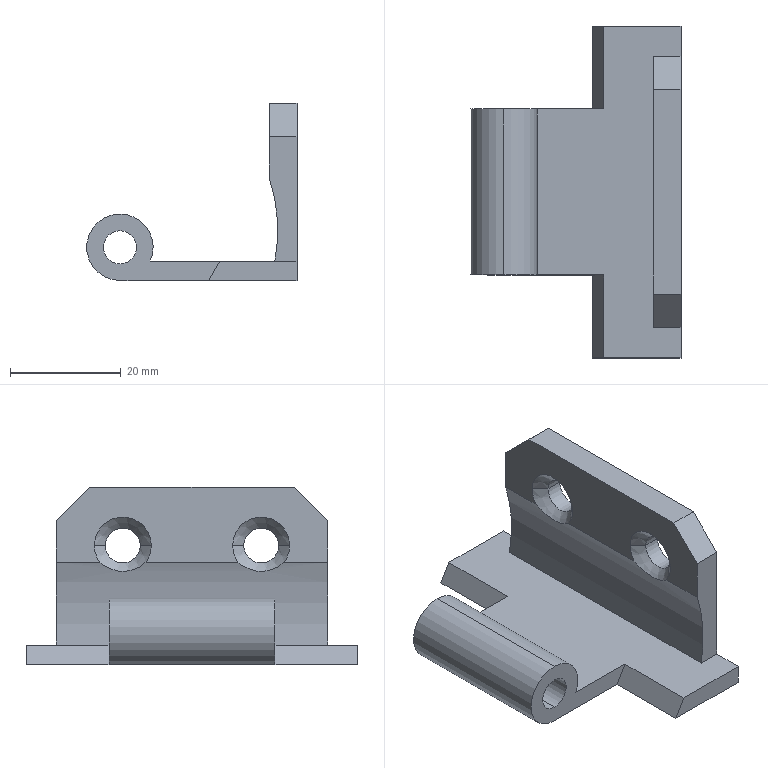Component | SolidWorks | SidePanelAssembly-1_GL213-1Hinge2-4 | 1 solid | 28 faces | box 38 x 60 x 32 mm | volume 12628 mm3 | plane 15 | cylinder 9 | cone 4 | commonest cylinder face diameters 6.3 x4 6 x2 12 x2 60 x1
build123d program:
from build123d import *

# Parameters (mm, degrees)
BOSS_EXTRUDE1_DEPTH = 60
SKETCH2_W           = 49
SKETCH2_H           = 5
BOSS_EXTRUDE2_DEPTH = 28.5
SKETCH3_W           = 3.5
SKETCH3_H           = 30
BOSS_EXTRUDE3_DEPTH = 27
SKETCH4_R           = 6
BOSS_EXTRUDE4_DEPTH = 30
SKETCH5_R           = 3
CUT_EXTRUDE1_DEPTH  = 30
SKETCH6_R           = 3.15
CUT_EXTRUDE2_DEPTH  = 30
CHAMFER1_SIZE       = 2
CHAMFER2_SIZE       = 6
CUT_EXTRUDE3_DEPTH  = 74.744


with BuildPart() as part:
    # Sketch1 → Boss-Extrude1 (new body)
    with BuildSketch(Plane.XY):
        Polygon((0, 0), (3.5, 0), (3.5, 13.979), (0, 16), align=None)
    extrude(amount=BOSS_EXTRUDE1_DEPTH)

    # Sketch2 → Boss-Extrude2 (add)
    with BuildSketch(Plane(origin=(3.5, 0, 0), x_dir=(0, 0, -1), z_dir=(1, 0, 0))):
        with Locations((-30, 2.5)):
            Rectangle(SKETCH2_W, SKETCH2_H)
    extrude(amount=BOSS_EXTRUDE2_DEPTH)

    # Sketch3 → Boss-Extrude3 (add)
    with BuildSketch(Plane(origin=(0, 5, 0), x_dir=(1, 0, 0), z_dir=(0, 1, 0))):
        with Locations((1.75, -30)):
            Rectangle(SKETCH3_W, SKETCH3_H)
    extrude(amount=BOSS_EXTRUDE3_DEPTH)

    # Sketch4 → Boss-Extrude4 (add)
    with BuildSketch(Plane.XY.offset(45)):
        with Locations((6, 32)):
            Circle(SKETCH4_R)
    extrude(amount=-BOSS_EXTRUDE4_DEPTH)

    # Sketch5 → Cut-Extrude1 (cut)
    with BuildSketch(Plane.XY.offset(45)):
        with Locations((6, 32)):
            Circle(SKETCH5_R)
    extrude(amount=-CUT_EXTRUDE1_DEPTH, mode=Mode.SUBTRACT)

    # Sketch6 → Cut-Extrude2 (cut)
    with BuildSketch(Plane(origin=(0, 5, 0), x_dir=(1, 0, 0), z_dir=(0, 1, 0))):
        with Locations(Location((21.5, -42.5, 0), (0, 0, 270))):
            Circle(SKETCH6_R)
        with Locations(Location((21.5, -17.5, 0), (0, 0, 270))):
            Circle(SKETCH6_R)
    extrude(amount=-CUT_EXTRUDE2_DEPTH, mode=Mode.SUBTRACT)

    # Chamfer1
    chamfer1_edges = [part.edges().sort_by_distance(p)[0] for p in [
        (21.5, 5, 39.35),
        (21.5, 5, 14.35),
    ]]
    chamfer(chamfer1_edges, length=CHAMFER1_SIZE)

    # Chamfer2
    chamfer2_edges = [part.edges().sort_by_distance(p)[0] for p in [
        (32, 2.5, 54.5),
        (32, 2.5, 5.5),
    ]]
    chamfer(chamfer2_edges, length=CHAMFER2_SIZE)

    # Sketch7 → Cut-Extrude3 (cut, through all)
    with BuildSketch(Plane.XY.offset(54.5)):
        with BuildLine():
            Line((3.5, 4), (3.5, 5))
            Line((3.5, 5), (18.5, 5))
            ThreePointArc((18.5, 5), (11.064, 3.545), (3.5, 4))
        make_face()
    extrude(amount=-CUT_EXTRUDE3_DEPTH, mode=Mode.SUBTRACT)


solid = part.part

# Placed as in the assembly
solid = solid.moved(Location((-417.218, 212.1, -600), (90, 0, 90)))
STEP:
#1=CARTESIAN_POINT('',(-16.544,7.785,-22.776));
#2=VERTEX_POINT('',#1);
#3=CARTESIAN_POINT('',(-16.544,7.537,-22.776));
#4=VERTEX_POINT('',#3);
#5=CARTESIAN_POINT('',(-16.544,7.661,-22.776));
#6=DIRECTION('',(-1.,-0.,-0.));
#7=DIRECTION('',(0.,1.,0.));
#8=AXIS2_PLACEMENT_3D('',#5,#6,#7);
#9=CIRCLE('',#8,0.124);
#10=EDGE_CURVE('',#2,#4,#9,.T.);
#11=ORIENTED_EDGE('',*,*,#10,.F.);
#12=CARTESIAN_POINT('',(-16.623,7.864,-22.776));
#13=VERTEX_POINT('',#12);
#14=CARTESIAN_POINT('',(-16.544,7.785,-22.776));
#15=DIRECTION('',(-0.7071,0.7071,-0.));
#16=VECTOR('',#15,39.37);
#17=LINE('',#14,#16);
#18=EDGE_CURVE('',#2,#13,#17,.T.);
#19=ORIENTED_EDGE('',*,*,#18,.T.);
#20=CARTESIAN_POINT('',(-16.623,7.826,-22.894));
#21=VERTEX_POINT('',#20);
#22=CARTESIAN_POINT('',(-16.623,7.661,-22.776));
#23=DIRECTION('',(1.,0.,0.));
#24=DIRECTION('',(0.,1.,0.));
#25=AXIS2_PLACEMENT_3D('',#22,#23,#24);
#26=CIRCLE('',#25,0.2028);
#27=EDGE_CURVE('',#21,#13,#26,.T.);
#28=ORIENTED_EDGE('',*,*,#27,.F.);
#29=CARTESIAN_POINT('',(-16.623,7.497,-22.894));
#30=VERTEX_POINT('',#29);
#31=CARTESIAN_POINT('',(-16.623,7.497,-22.894));
#32=CARTESIAN_POINT('',(-16.619,7.508,-22.904));
#33=CARTESIAN_POINT('',(-16.617,7.52,-22.913));
#34=CARTESIAN_POINT('',(-16.613,7.538,-22.925));
#35=CARTESIAN_POINT('',(-16.612,7.545,-22.928));
#36=CARTESIAN_POINT('',(-16.61,7.558,-22.935));
#37=CARTESIAN_POINT('',(-16.609,7.565,-22.938));
#38=CARTESIAN_POINT('',(-16.606,7.586,-22.947));
#39=CARTESIAN_POINT('',(-16.605,7.601,-22.951));
#40=CARTESIAN_POINT('',(-16.604,7.623,-22.956));
#41=CARTESIAN_POINT('',(-16.604,7.631,-22.957));
#42=CARTESIAN_POINT('',(-16.603,7.646,-22.958));
#43=CARTESIAN_POINT('',(-16.603,7.653,-22.959));
#44=CARTESIAN_POINT('',(-16.603,7.676,-22.959));
#45=CARTESIAN_POINT('',(-16.604,7.691,-22.957));
#46=CARTESIAN_POINT('',(-16.605,7.721,-22.952));
#47=CARTESIAN_POINT('',(-16.606,7.736,-22.947));
#48=CARTESIAN_POINT('',(-16.61,7.764,-22.936));
#49=CARTESIAN_POINT('',(-16.612,7.777,-22.929));
#50=CARTESIAN_POINT('',(-16.617,7.803,-22.913));
#51=CARTESIAN_POINT('',(-16.619,7.815,-22.904));
#52=CARTESIAN_POINT('',(-16.623,7.826,-22.894));
#53=B_SPLINE_CURVE_WITH_KNOTS('',3,(#31,#32,#33,#34,#35,#36,#37,#38,#39,#40,#41,#42,#43,#44,#45,#46,#47,#48,#49,#50,#51,#52),.UNSPECIFIED.,.F.,.F.,(4,2,2,2,2,2,2,2,2,2,4),(0.0003209,0.001473,0.002049,0.002625,0.003777,0.004353,0.00493,0.006082,0.007234,0.008386,0.009538),.UNSPECIFIED.);
#54=EDGE_CURVE('',#30,#21,#53,.T.);
#55=ORIENTED_EDGE('',*,*,#54,.F.);
#56=CARTESIAN_POINT('',(-16.623,7.459,-22.776));
#57=VERTEX_POINT('',#56);
#58=CARTESIAN_POINT('',(-16.623,7.661,-22.776));
#59=DIRECTION('',(1.,0.,0.));
#60=DIRECTION('',(0.,1.,0.));
#61=AXIS2_PLACEMENT_3D('',#58,#59,#60);
#62=CIRCLE('',#61,0.2028);
#63=EDGE_CURVE('',#57,#30,#62,.T.);
#64=ORIENTED_EDGE('',*,*,#63,.F.);
#65=CARTESIAN_POINT('',(-16.544,7.537,-22.776));
#66=DIRECTION('',(-0.7071,-0.7071,-0.));
#67=VECTOR('',#66,39.37);
#68=LINE('',#65,#67);
#69=EDGE_CURVE('',#4,#57,#68,.T.);
#70=ORIENTED_EDGE('',*,*,#69,.F.);
#71=EDGE_LOOP('',(#11,#19,#28,#55,#64,#70));
#72=FACE_OUTER_BOUND('',#71,.T.);
#73=CARTESIAN_POINT('',(-16.544,7.661,-22.776));
#74=DIRECTION('',(-1.,-0.,-0.));
#75=DIRECTION('',(0.,-1.,0.));
#76=AXIS2_PLACEMENT_3D('',#73,#74,#75);
#77=CONICAL_SURFACE('',#76,0.124,0.7854);
#78=ADVANCED_FACE('',(#72),#77,.F.);
#79=CARTESIAN_POINT('',(-16.544,6.801,-22.776));
#80=VERTEX_POINT('',#79);
#81=CARTESIAN_POINT('',(-16.544,6.553,-22.776));
#82=VERTEX_POINT('',#81);
#83=CARTESIAN_POINT('',(-16.544,6.677,-22.776));
#84=DIRECTION('',(-1.,-0.,-0.));
#85=DIRECTION('',(0.,1.,0.));
#86=AXIS2_PLACEMENT_3D('',#83,#84,#85);
#87=CIRCLE('',#86,0.124);
#88=EDGE_CURVE('',#80,#82,#87,.T.);
#89=ORIENTED_EDGE('',*,*,#88,.F.);
#90=CARTESIAN_POINT('',(-16.623,6.88,-22.776));
#91=VERTEX_POINT('',#90);
#92=CARTESIAN_POINT('',(-16.544,6.801,-22.776));
#93=DIRECTION('',(-0.7071,0.7071,-0.));
#94=VECTOR('',#93,39.37);
#95=LINE('',#92,#94);
#96=EDGE_CURVE('',#80,#91,#95,.T.);
#97=ORIENTED_EDGE('',*,*,#96,.T.);
#98=CARTESIAN_POINT('',(-16.623,6.842,-22.894));
#99=VERTEX_POINT('',#98);
#100=CARTESIAN_POINT('',(-16.623,6.677,-22.776));
#101=DIRECTION('',(1.,0.,0.));
#102=DIRECTION('',(0.,1.,0.));
#103=AXIS2_PLACEMENT_3D('',#100,#101,#102);
#104=CIRCLE('',#103,0.2028);
#105=EDGE_CURVE('',#99,#91,#104,.T.);
#106=ORIENTED_EDGE('',*,*,#105,.F.);
#107=CARTESIAN_POINT('',(-16.623,6.512,-22.894));
#108=VERTEX_POINT('',#107);
#109=CARTESIAN_POINT('',(-16.623,6.512,-22.894));
#110=CARTESIAN_POINT('',(-16.619,6.523,-22.904));
#111=CARTESIAN_POINT('',(-16.617,6.535,-22.913));
#112=CARTESIAN_POINT('',(-16.613,6.554,-22.925));
#113=CARTESIAN_POINT('',(-16.612,6.561,-22.928));
#114=CARTESIAN_POINT('',(-16.61,6.574,-22.935));
#115=CARTESIAN_POINT('',(-16.609,6.581,-22.938));
#116=CARTESIAN_POINT('',(-16.606,6.602,-22.947));
#117=CARTESIAN_POINT('',(-16.605,6.617,-22.951));
#118=CARTESIAN_POINT('',(-16.604,6.639,-22.956));
#119=CARTESIAN_POINT('',(-16.604,6.646,-22.957));
#120=CARTESIAN_POINT('',(-16.603,6.661,-22.958));
#121=CARTESIAN_POINT('',(-16.603,6.669,-22.959));
#122=CARTESIAN_POINT('',(-16.603,6.692,-22.959));
#123=CARTESIAN_POINT('',(-16.604,6.707,-22.957));
#124=CARTESIAN_POINT('',(-16.605,6.737,-22.952));
#125=CARTESIAN_POINT('',(-16.606,6.752,-22.947));
#126=CARTESIAN_POINT('',(-16.61,6.78,-22.936));
#127=CARTESIAN_POINT('',(-16.612,6.793,-22.929));
#128=CARTESIAN_POINT('',(-16.617,6.819,-22.913));
#129=CARTESIAN_POINT('',(-16.619,6.831,-22.904));
#130=CARTESIAN_POINT('',(-16.623,6.842,-22.894));
#131=B_SPLINE_CURVE_WITH_KNOTS('',3,(#109,#110,#111,#112,#113,#114,#115,#116,#117,#118,#119,#120,#121,#122,#123,#124,#125,#126,#127,#128,#129,#130),.UNSPECIFIED.,.F.,.F.,(4,2,2,2,2,2,2,2,2,2,4),(0.0003209,0.001473,0.002049,0.002625,0.003777,0.004353,0.00493,0.006082,0.007234,0.008386,0.009538),.UNSPECIFIED.);
#132=EDGE_CURVE('',#108,#99,#131,.T.);
#133=ORIENTED_EDGE('',*,*,#132,.F.);
#134=CARTESIAN_POINT('',(-16.623,6.474,-22.776));
#135=VERTEX_POINT('',#134);
#136=CARTESIAN_POINT('',(-16.623,6.677,-22.776));
#137=DIRECTION('',(1.,0.,0.));
#138=DIRECTION('',(0.,1.,0.));
#139=AXIS2_PLACEMENT_3D('',#136,#137,#138);
#140=CIRCLE('',#139,0.2028);
#141=EDGE_CURVE('',#135,#108,#140,.T.);
#142=ORIENTED_EDGE('',*,*,#141,.F.);
#143=CARTESIAN_POINT('',(-16.544,6.553,-22.776));
#144=DIRECTION('',(-0.7071,-0.7071,-0.));
#145=VECTOR('',#144,39.37);
#146=LINE('',#143,#145);
#147=EDGE_CURVE('',#82,#135,#146,.T.);
#148=ORIENTED_EDGE('',*,*,#147,.F.);
#149=EDGE_LOOP('',(#89,#97,#106,#133,#142,#148));
#150=FACE_OUTER_BOUND('',#149,.T.);
#151=CARTESIAN_POINT('',(-16.544,6.677,-22.776));
#152=DIRECTION('',(-1.,-0.,-0.));
#153=DIRECTION('',(0.,-1.,0.));
#154=AXIS2_PLACEMENT_3D('',#151,#152,#153);
#155=CONICAL_SURFACE('',#154,0.124,0.7854);
#156=ADVANCED_FACE('',(#150),#155,.F.);
#157=CARTESIAN_POINT('',(-16.426,7.785,-22.776));
#158=VERTEX_POINT('',#157);
#159=CARTESIAN_POINT('',(-16.426,7.537,-22.776));
#160=VERTEX_POINT('',#159);
#161=CARTESIAN_POINT('',(-16.426,7.661,-22.776));
#162=DIRECTION('',(-1.,-0.,-0.));
#163=DIRECTION('',(0.,-1.,0.));
#164=AXIS2_PLACEMENT_3D('',#161,#162,#163);
#165=CIRCLE('',#164,0.124);
#166=EDGE_CURVE('',#158,#160,#165,.T.);
#167=ORIENTED_EDGE('',*,*,#166,.F.);
#168=CARTESIAN_POINT('',(-15.442,7.785,-22.776));
#169=DIRECTION('',(-1.,-0.,-0.));
#170=VECTOR('',#169,39.37);
#171=LINE('',#168,#170);
#172=EDGE_CURVE('',#158,#2,#171,.T.);
#173=ORIENTED_EDGE('',*,*,#172,.T.);
#174=ORIENTED_EDGE('',*,*,#10,.T.);
#175=CARTESIAN_POINT('',(-15.442,7.537,-22.776));
#176=DIRECTION('',(-1.,-0.,-0.));
#177=VECTOR('',#176,39.37);
#178=LINE('',#175,#177);
#179=EDGE_CURVE('',#160,#4,#178,.T.);
#180=ORIENTED_EDGE('',*,*,#179,.F.);
#181=EDGE_LOOP('',(#167,#173,#174,#180));
#182=FACE_OUTER_BOUND('',#181,.T.);
#183=CARTESIAN_POINT('',(-15.442,7.661,-22.776));
#184=DIRECTION('',(-1.,-0.,-0.));
#185=DIRECTION('',(0.,-1.,0.));
#186=AXIS2_PLACEMENT_3D('',#183,#184,#185);
#187=CYLINDRICAL_SURFACE('',#186,0.124);
#188=ADVANCED_FACE('',(#182),#187,.F.);
#189=CARTESIAN_POINT('',(-16.426,6.801,-22.776));
#190=VERTEX_POINT('',#189);
#191=CARTESIAN_POINT('',(-16.426,6.553,-22.776));
#192=VERTEX_POINT('',#191);
#193=CARTESIAN_POINT('',(-16.426,6.677,-22.776));
#194=DIRECTION('',(-1.,-0.,-0.));
#195=DIRECTION('',(0.,-1.,0.));
#196=AXIS2_PLACEMENT_3D('',#193,#194,#195);
#197=CIRCLE('',#196,0.124);
#198=EDGE_CURVE('',#190,#192,#197,.T.);
#199=ORIENTED_EDGE('',*,*,#198,.F.);
#200=CARTESIAN_POINT('',(-15.442,6.801,-22.776));
#201=DIRECTION('',(-1.,-0.,-0.));
#202=VECTOR('',#201,39.37);
#203=LINE('',#200,#202);
#204=EDGE_CURVE('',#190,#80,#203,.T.);
#205=ORIENTED_EDGE('',*,*,#204,.T.);
#206=ORIENTED_EDGE('',*,*,#88,.T.);
#207=CARTESIAN_POINT('',(-15.442,6.553,-22.776));
#208=DIRECTION('',(-1.,-0.,-0.));
#209=VECTOR('',#208,39.37);
#210=LINE('',#207,#209);
#211=EDGE_CURVE('',#192,#82,#210,.T.);
#212=ORIENTED_EDGE('',*,*,#211,.F.);
#213=EDGE_LOOP('',(#199,#205,#206,#212));
#214=FACE_OUTER_BOUND('',#213,.T.);
#215=CARTESIAN_POINT('',(-15.442,6.677,-22.776));
#216=DIRECTION('',(-1.,-0.,-0.));
#217=DIRECTION('',(0.,-1.,0.));
#218=AXIS2_PLACEMENT_3D('',#215,#216,#217);
#219=CYLINDRICAL_SURFACE('',#218,0.124);
#220=ADVANCED_FACE('',(#214),#219,.F.);
#221=CARTESIAN_POINT('',(-17.686,7.76,-23.504));
#222=VERTEX_POINT('',#221);
#223=CARTESIAN_POINT('',(-17.686,7.76,-23.268));
#224=VERTEX_POINT('',#223);
#225=CARTESIAN_POINT('',(-17.686,7.76,-23.386));
#226=DIRECTION('',(0.,-1.,-0.));
#227=DIRECTION('',(0.,0.,1.));
#228=AXIS2_PLACEMENT_3D('',#225,#226,#227);
#229=CIRCLE('',#228,0.1181);
#230=EDGE_CURVE('',#222,#224,#229,.T.);
#231=ORIENTED_EDGE('',*,*,#230,.F.);
#232=CARTESIAN_POINT('',(-17.686,6.579,-23.504));
#233=VERTEX_POINT('',#232);
#234=CARTESIAN_POINT('',(-17.686,7.76,-23.504));
#235=DIRECTION('',(0.,-1.,-0.));
#236=VECTOR('',#235,39.37);
#237=LINE('',#234,#236);
#238=EDGE_CURVE('',#222,#233,#237,.T.);
#239=ORIENTED_EDGE('',*,*,#238,.T.);
#240=CARTESIAN_POINT('',(-17.686,6.579,-23.268));
#241=VERTEX_POINT('',#240);
#242=CARTESIAN_POINT('',(-17.686,6.579,-23.386));
#243=DIRECTION('',(0.,-1.,-0.));
#244=DIRECTION('',(0.,0.,1.));
#245=AXIS2_PLACEMENT_3D('',#242,#243,#244);
#246=CIRCLE('',#245,0.1181);
#247=EDGE_CURVE('',#233,#241,#246,.T.);
#248=ORIENTED_EDGE('',*,*,#247,.T.);
#249=CARTESIAN_POINT('',(-17.686,7.76,-23.268));
#250=DIRECTION('',(0.,-1.,-0.));
#251=VECTOR('',#250,39.37);
#252=LINE('',#249,#251);
#253=EDGE_CURVE('',#224,#241,#252,.T.);
#254=ORIENTED_EDGE('',*,*,#253,.F.);
#255=EDGE_LOOP('',(#231,#239,#248,#254));
#256=FACE_OUTER_BOUND('',#255,.T.);
#257=CARTESIAN_POINT('',(-17.686,7.76,-23.386));
#258=DIRECTION('',(0.,-1.,-0.));
#259=DIRECTION('',(0.,0.,1.));
#260=AXIS2_PLACEMENT_3D('',#257,#258,#259);
#261=CYLINDRICAL_SURFACE('',#260,0.1181);
#262=ADVANCED_FACE('',(#256),#261,.F.);
#263=CARTESIAN_POINT('',(-17.471,7.76,-23.484));
#264=VERTEX_POINT('',#263);
#265=CARTESIAN_POINT('',(-17.686,7.76,-23.15));
#266=VERTEX_POINT('',#265);
#267=CARTESIAN_POINT('',(-17.686,7.76,-23.386));
#268=DIRECTION('',(0.,-1.,-0.));
#269=DIRECTION('',(0.,0.,1.));
#270=AXIS2_PLACEMENT_3D('',#267,#268,#269);
#271=CIRCLE('',#270,0.2362);
#272=EDGE_CURVE('',#264,#266,#271,.T.);
#273=ORIENTED_EDGE('',*,*,#272,.T.);
#274=CARTESIAN_POINT('',(-17.686,6.579,-23.15));
#275=VERTEX_POINT('',#274);
#276=CARTESIAN_POINT('',(-17.686,7.76,-23.15));
#277=DIRECTION('',(0.,-1.,-0.));
#278=VECTOR('',#277,39.37);
#279=LINE('',#276,#278);
#280=EDGE_CURVE('',#266,#275,#279,.T.);
#281=ORIENTED_EDGE('',*,*,#280,.T.);
#282=CARTESIAN_POINT('',(-17.471,6.579,-23.484));
#283=VERTEX_POINT('',#282);
#284=CARTESIAN_POINT('',(-17.686,6.579,-23.386));
#285=DIRECTION('',(0.,-1.,-0.));
#286=DIRECTION('',(0.,0.,1.));
#287=AXIS2_PLACEMENT_3D('',#284,#285,#286);
#288=CIRCLE('',#287,0.2362);
#289=EDGE_CURVE('',#283,#275,#288,.T.);
#290=ORIENTED_EDGE('',*,*,#289,.F.);
#291=CARTESIAN_POINT('',(-17.471,7.76,-23.484));
#292=DIRECTION('',(0.,-1.,-0.));
#293=VECTOR('',#292,39.37);
#294=LINE('',#291,#293);
#295=EDGE_CURVE('',#264,#283,#294,.T.);
#296=ORIENTED_EDGE('',*,*,#295,.F.);
#297=EDGE_LOOP('',(#273,#281,#290,#296));
#298=FACE_OUTER_BOUND('',#297,.T.);
#299=CARTESIAN_POINT('',(-17.686,7.76,-23.386));
#300=DIRECTION('',(0.,-1.,-0.));
#301=DIRECTION('',(0.,0.,1.));
#302=AXIS2_PLACEMENT_3D('',#299,#300,#301);
#303=CYLINDRICAL_SURFACE('',#302,0.2362);
#304=ADVANCED_FACE('',(#298),#303,.T.);
#305=CARTESIAN_POINT('',(-17.056,6.579,-23.622));
#306=VERTEX_POINT('',#305);
#307=CARTESIAN_POINT('',(-16.976,6.579,-23.484));
#308=VERTEX_POINT('',#307);
#309=CARTESIAN_POINT('',(-16.976,6.579,-23.484));
#310=DIRECTION('',(0.5,-0.,0.866));
#311=VECTOR('',#310,39.37);
#312=LINE('',#309,#311);
#313=EDGE_CURVE('',#306,#308,#312,.T.);
#314=ORIENTED_EDGE('',*,*,#313,.F.);
#315=CARTESIAN_POINT('',(-17.056,5.988,-23.622));
#316=VERTEX_POINT('',#315);
#317=CARTESIAN_POINT('',(-17.056,5.988,-23.622));
#318=DIRECTION('',(-0.,1.,0.));
#319=VECTOR('',#318,39.37);
#320=LINE('',#317,#319);
#321=EDGE_CURVE('',#316,#306,#320,.T.);
#322=ORIENTED_EDGE('',*,*,#321,.F.);
#323=CARTESIAN_POINT('',(-16.976,5.988,-23.484));
#324=VERTEX_POINT('',#323);
#325=CARTESIAN_POINT('',(-16.976,5.988,-23.484));
#326=DIRECTION('',(-0.5,0.,-0.866));
#327=VECTOR('',#326,39.37);
#328=LINE('',#325,#327);
#329=EDGE_CURVE('',#324,#316,#328,.T.);
#330=ORIENTED_EDGE('',*,*,#329,.F.);
#331=CARTESIAN_POINT('',(-16.976,5.988,-23.484));
#332=DIRECTION('',(-0.,1.,0.));
#333=VECTOR('',#332,39.37);
#334=LINE('',#331,#333);
#335=EDGE_CURVE('',#324,#308,#334,.T.);
#336=ORIENTED_EDGE('',*,*,#335,.T.);
#337=EDGE_LOOP('',(#314,#322,#330,#336));
#338=FACE_OUTER_BOUND('',#337,.T.);
#339=CARTESIAN_POINT('',(-16.976,5.988,-23.484));
#340=DIRECTION('',(0.866,0.,-0.5));
#341=DIRECTION('',(0.5,-0.,0.866));
#342=AXIS2_PLACEMENT_3D('',#339,#340,#341);
#343=PLANE('',#342);
#344=ADVANCED_FACE('',(#338),#343,.F.);
#345=CARTESIAN_POINT('',(-16.976,7.76,-23.484));
#346=VERTEX_POINT('',#345);
#347=CARTESIAN_POINT('',(-17.056,7.76,-23.622));
#348=VERTEX_POINT('',#347);
#349=CARTESIAN_POINT('',(-16.976,7.76,-23.484));
#350=DIRECTION('',(-0.5,0.,-0.866));
#351=VECTOR('',#350,39.37);
#352=LINE('',#349,#351);
#353=EDGE_CURVE('',#346,#348,#352,.T.);
#354=ORIENTED_EDGE('',*,*,#353,.F.);
#355=CARTESIAN_POINT('',(-16.976,8.35,-23.484));
#356=VERTEX_POINT('',#355);
#357=CARTESIAN_POINT('',(-16.976,5.988,-23.484));
#358=DIRECTION('',(-0.,1.,0.));
#359=VECTOR('',#358,39.37);
#360=LINE('',#357,#359);
#361=EDGE_CURVE('',#346,#356,#360,.T.);
#362=ORIENTED_EDGE('',*,*,#361,.T.);
#363=CARTESIAN_POINT('',(-17.056,8.35,-23.622));
#364=VERTEX_POINT('',#363);
#365=CARTESIAN_POINT('',(-16.976,8.35,-23.484));
#366=DIRECTION('',(-0.5,0.,-0.866));
#367=VECTOR('',#366,39.37);
#368=LINE('',#365,#367);
#369=EDGE_CURVE('',#356,#364,#368,.T.);
#370=ORIENTED_EDGE('',*,*,#369,.T.);
#371=CARTESIAN_POINT('',(-17.056,5.988,-23.622));
#372=DIRECTION('',(-0.,1.,0.));
#373=VECTOR('',#372,39.37);
#374=LINE('',#371,#373);
#375=EDGE_CURVE('',#348,#364,#374,.T.);
#376=ORIENTED_EDGE('',*,*,#375,.F.);
#377=EDGE_LOOP('',(#354,#362,#370,#376));
#378=FACE_OUTER_BOUND('',#377,.T.);
#379=CARTESIAN_POINT('',(-16.976,5.988,-23.484));
#380=DIRECTION('',(0.866,0.,-0.5));
#381=DIRECTION('',(0.5,-0.,0.866));
#382=AXIS2_PLACEMENT_3D('',#379,#380,#381);
#383=PLANE('',#382);
#384=ADVANCED_FACE('',(#378),#383,.F.);
#385=CARTESIAN_POINT('',(-16.426,8.35,-23.484));
#386=VERTEX_POINT('',#385);
#387=CARTESIAN_POINT('',(-16.426,8.35,-23.484));
#388=DIRECTION('',(-1.,-0.,-0.));
#389=VECTOR('',#388,39.37);
#390=LINE('',#387,#389);
#391=EDGE_CURVE('',#386,#356,#390,.T.);
#392=ORIENTED_EDGE('',*,*,#391,.T.);
#393=ORIENTED_EDGE('',*,*,#361,.F.);
#394=CARTESIAN_POINT('',(-17.686,7.76,-23.484));
#395=DIRECTION('',(1.,0.,0.));
#396=VECTOR('',#395,39.37);
#397=LINE('',#394,#396);
#398=EDGE_CURVE('',#264,#346,#397,.T.);
#399=ORIENTED_EDGE('',*,*,#398,.F.);
#400=ORIENTED_EDGE('',*,*,#295,.T.);
#401=CARTESIAN_POINT('',(-17.686,6.579,-23.484));
#402=DIRECTION('',(1.,0.,0.));
#403=VECTOR('',#402,39.37);
#404=LINE('',#401,#403);
#405=EDGE_CURVE('',#283,#308,#404,.T.);
#406=ORIENTED_EDGE('',*,*,#405,.T.);
#407=ORIENTED_EDGE('',*,*,#335,.F.);
#408=CARTESIAN_POINT('',(-16.426,5.988,-23.484));
#409=VERTEX_POINT('',#408);
#410=CARTESIAN_POINT('',(-16.426,5.988,-23.484));
#411=DIRECTION('',(-1.,-0.,-0.));
#412=VECTOR('',#411,39.37);
#413=LINE('',#410,#412);
#414=EDGE_CURVE('',#409,#324,#413,.T.);
#415=ORIENTED_EDGE('',*,*,#414,.F.);
#416=CARTESIAN_POINT('',(-16.426,6.205,-23.484));
#417=VERTEX_POINT('',#416);
#418=CARTESIAN_POINT('',(-16.426,5.988,-23.484));
#419=DIRECTION('',(-0.,1.,0.));
#420=VECTOR('',#419,39.37);
#421=LINE('',#418,#420);
#422=EDGE_CURVE('',#409,#417,#421,.T.);
#423=ORIENTED_EDGE('',*,*,#422,.T.);
#424=CARTESIAN_POINT('',(-16.583,6.205,-23.484));
#425=VERTEX_POINT('',#424);
#426=CARTESIAN_POINT('',(-16.426,6.205,-23.484));
#427=DIRECTION('',(1.,0.,0.));
#428=VECTOR('',#427,39.37);
#429=LINE('',#426,#428);
#430=EDGE_CURVE('',#425,#417,#429,.T.);
#431=ORIENTED_EDGE('',*,*,#430,.F.);
#432=CARTESIAN_POINT('',(-16.583,8.134,-23.484));
#433=VERTEX_POINT('',#432);
#434=CARTESIAN_POINT('',(-16.583,8.35,-23.484));
#435=DIRECTION('',(0.,-1.,-0.));
#436=VECTOR('',#435,39.37);
#437=LINE('',#434,#436);
#438=EDGE_CURVE('',#433,#425,#437,.T.);
#439=ORIENTED_EDGE('',*,*,#438,.F.);
#440=CARTESIAN_POINT('',(-16.426,8.134,-23.484));
#441=VERTEX_POINT('',#440);
#442=CARTESIAN_POINT('',(-16.426,8.134,-23.484));
#443=DIRECTION('',(-1.,-0.,-0.));
#444=VECTOR('',#443,39.37);
#445=LINE('',#442,#444);
#446=EDGE_CURVE('',#441,#433,#445,.T.);
#447=ORIENTED_EDGE('',*,*,#446,.F.);
#448=CARTESIAN_POINT('',(-16.426,5.988,-23.484));
#449=DIRECTION('',(-0.,1.,0.));
#450=VECTOR('',#449,39.37);
#451=LINE('',#448,#450);
#452=EDGE_CURVE('',#441,#386,#451,.T.);
#453=ORIENTED_EDGE('',*,*,#452,.T.);
#454=EDGE_LOOP('',(#392,#393,#399,#400,#406,#407,#415,#423,#431,#439,#447,#453));
#455=FACE_OUTER_BOUND('',#454,.T.);
#456=CARTESIAN_POINT('',(-16.426,5.988,-23.484));
#457=DIRECTION('',(0.,0.,-1.));
#458=DIRECTION('',(0.,-1.,-0.));
#459=AXIS2_PLACEMENT_3D('',#456,#457,#458);
#460=PLANE('',#459);
#461=ADVANCED_FACE('',(#455),#460,.F.);
#462=ORIENTED_EDGE('',*,*,#321,.T.);
#463=CARTESIAN_POINT('',(-17.686,6.579,-23.622));
#464=VERTEX_POINT('',#463);
#465=CARTESIAN_POINT('',(-17.686,6.579,-23.622));
#466=DIRECTION('',(1.,0.,0.));
#467=VECTOR('',#466,39.37);
#468=LINE('',#465,#467);
#469=EDGE_CURVE('',#464,#306,#468,.T.);
#470=ORIENTED_EDGE('',*,*,#469,.F.);
#471=CARTESIAN_POINT('',(-17.686,7.76,-23.622));
#472=VERTEX_POINT('',#471);
#473=CARTESIAN_POINT('',(-17.686,7.76,-23.622));
#474=DIRECTION('',(0.,-1.,-0.));
#475=VECTOR('',#474,39.37);
#476=LINE('',#473,#475);
#477=EDGE_CURVE('',#472,#464,#476,.T.);
#478=ORIENTED_EDGE('',*,*,#477,.F.);
#479=CARTESIAN_POINT('',(-17.686,7.76,-23.622));
#480=DIRECTION('',(1.,0.,0.));
#481=VECTOR('',#480,39.37);
#482=LINE('',#479,#481);
#483=EDGE_CURVE('',#472,#348,#482,.T.);
#484=ORIENTED_EDGE('',*,*,#483,.T.);
#485=ORIENTED_EDGE('',*,*,#375,.T.);
#486=CARTESIAN_POINT('',(-16.426,8.35,-23.622));
#487=VERTEX_POINT('',#486);
#488=CARTESIAN_POINT('',(-17.056,8.35,-23.622));
#489=DIRECTION('',(1.,0.,0.));
#490=VECTOR('',#489,39.37);
#491=LINE('',#488,#490);
#492=EDGE_CURVE('',#364,#487,#491,.T.);
#493=ORIENTED_EDGE('',*,*,#492,.T.);
#494=CARTESIAN_POINT('',(-16.426,5.988,-23.622));
#495=VERTEX_POINT('',#494);
#496=CARTESIAN_POINT('',(-16.426,5.988,-23.622));
#497=DIRECTION('',(-0.,1.,0.));
#498=VECTOR('',#497,39.37);
#499=LINE('',#496,#498);
#500=EDGE_CURVE('',#495,#487,#499,.T.);
#501=ORIENTED_EDGE('',*,*,#500,.F.);
#502=CARTESIAN_POINT('',(-17.056,5.988,-23.622));
#503=DIRECTION('',(1.,0.,0.));
#504=VECTOR('',#503,39.37);
#505=LINE('',#502,#504);
#506=EDGE_CURVE('',#316,#495,#505,.T.);
#507=ORIENTED_EDGE('',*,*,#506,.F.);
#508=EDGE_LOOP('',(#462,#470,#478,#484,#485,#493,#501,#507));
#509=FACE_OUTER_BOUND('',#508,.T.);
#510=CARTESIAN_POINT('',(-17.056,5.988,-23.622));
#511=DIRECTION('',(-0.,-0.,1.));
#512=DIRECTION('',(-1.,-0.,-0.));
#513=AXIS2_PLACEMENT_3D('',#510,#511,#512);
#514=PLANE('',#513);
#515=ADVANCED_FACE('',(#509),#514,.F.);
#516=CARTESIAN_POINT('',(-16.426,7.661,-22.776));
#517=DIRECTION('',(-1.,-0.,-0.));
#518=DIRECTION('',(0.,-1.,0.));
#519=AXIS2_PLACEMENT_3D('',#516,#517,#518);
#520=CIRCLE('',#519,0.124);
#521=EDGE_CURVE('',#160,#158,#520,.T.);
#522=ORIENTED_EDGE('',*,*,#521,.T.);
#523=ORIENTED_EDGE('',*,*,#166,.T.);
#524=EDGE_LOOP('',(#522,#523));
#525=FACE_BOUND('',#524,.T.);
#526=CARTESIAN_POINT('',(-16.426,6.677,-22.776));
#527=DIRECTION('',(-1.,-0.,-0.));
#528=DIRECTION('',(0.,-1.,0.));
#529=AXIS2_PLACEMENT_3D('',#526,#527,#528);
#530=CIRCLE('',#529,0.124);
#531=EDGE_CURVE('',#192,#190,#530,.T.);
#532=ORIENTED_EDGE('',*,*,#531,.T.);
#533=ORIENTED_EDGE('',*,*,#198,.T.);
#534=EDGE_LOOP('',(#532,#533));
#535=FACE_BOUND('',#534,.T.);
#536=CARTESIAN_POINT('',(-16.426,6.441,-22.362));
#537=VERTEX_POINT('',#536);
#538=CARTESIAN_POINT('',(-16.426,7.898,-22.362));
#539=VERTEX_POINT('',#538);
#540=CARTESIAN_POINT('',(-16.426,6.205,-22.362));
#541=DIRECTION('',(-0.,1.,0.));
#542=VECTOR('',#541,39.37);
#543=LINE('',#540,#542);
#544=EDGE_CURVE('',#537,#539,#543,.T.);
#545=ORIENTED_EDGE('',*,*,#544,.F.);
#546=CARTESIAN_POINT('',(-16.426,6.205,-22.598));
#547=VERTEX_POINT('',#546);
#548=CARTESIAN_POINT('',(-16.426,6.441,-22.362));
#549=DIRECTION('',(0.,-0.7071,-0.7071));
#550=VECTOR('',#549,39.37);
#551=LINE('',#548,#550);
#552=EDGE_CURVE('',#537,#547,#551,.T.);
#553=ORIENTED_EDGE('',*,*,#552,.T.);
#554=CARTESIAN_POINT('',(-16.426,6.205,-22.362));
#555=DIRECTION('',(0.,0.,-1.));
#556=VECTOR('',#555,39.37);
#557=LINE('',#554,#556);
#558=EDGE_CURVE('',#547,#417,#557,.T.);
#559=ORIENTED_EDGE('',*,*,#558,.T.);
#560=ORIENTED_EDGE('',*,*,#422,.F.);
#561=CARTESIAN_POINT('',(-16.426,5.988,-23.622));
#562=DIRECTION('',(-0.,-0.,1.));
#563=VECTOR('',#562,39.37);
#564=LINE('',#561,#563);
#565=EDGE_CURVE('',#495,#409,#564,.T.);
#566=ORIENTED_EDGE('',*,*,#565,.F.);
#567=ORIENTED_EDGE('',*,*,#500,.T.);
#568=CARTESIAN_POINT('',(-16.426,8.35,-23.622));
#569=DIRECTION('',(-0.,-0.,1.));
#570=VECTOR('',#569,39.37);
#571=LINE('',#568,#570);
#572=EDGE_CURVE('',#487,#386,#571,.T.);
#573=ORIENTED_EDGE('',*,*,#572,.T.);
#574=ORIENTED_EDGE('',*,*,#452,.F.);
#575=CARTESIAN_POINT('',(-16.426,8.134,-22.598));
#576=VERTEX_POINT('',#575);
#577=CARTESIAN_POINT('',(-16.426,8.134,-22.362));
#578=DIRECTION('',(0.,0.,-1.));
#579=VECTOR('',#578,39.37);
#580=LINE('',#577,#579);
#581=EDGE_CURVE('',#576,#441,#580,.T.);
#582=ORIENTED_EDGE('',*,*,#581,.F.);
#583=CARTESIAN_POINT('',(-16.426,7.898,-22.362));
#584=DIRECTION('',(-0.,-0.7071,0.7071));
#585=VECTOR('',#584,39.37);
#586=LINE('',#583,#585);
#587=EDGE_CURVE('',#576,#539,#586,.T.);
#588=ORIENTED_EDGE('',*,*,#587,.T.);
#589=EDGE_LOOP('',(#545,#553,#559,#560,#566,#567,#573,#574,#582,#588));
#590=FACE_OUTER_BOUND('',#589,.T.);
#591=CARTESIAN_POINT('',(-16.426,5.988,-23.622));
#592=DIRECTION('',(-1.,-0.,-0.));
#593=DIRECTION('',(0.,-1.,-0.));
#594=AXIS2_PLACEMENT_3D('',#591,#592,#593);
#595=PLANE('',#594);
#596=ADVANCED_FACE('',(#525,#535,#590),#595,.F.);
#597=ORIENTED_EDGE('',*,*,#506,.T.);
#598=ORIENTED_EDGE('',*,*,#565,.T.);
#599=ORIENTED_EDGE('',*,*,#414,.T.);
#600=ORIENTED_EDGE('',*,*,#329,.T.);
#601=EDGE_LOOP('',(#597,#598,#599,#600));
#602=FACE_OUTER_BOUND('',#601,.T.);
#603=CARTESIAN_POINT('',(-16.426,5.988,-23.622));
#604=DIRECTION('',(0.,-1.,-0.));
#605=DIRECTION('',(-0.,-0.,1.));
#606=AXIS2_PLACEMENT_3D('',#603,#604,#605);
#607=PLANE('',#606);
#608=ADVANCED_FACE('',(#602),#607,.T.);
#609=ORIENTED_EDGE('',*,*,#492,.F.);
#610=ORIENTED_EDGE('',*,*,#369,.F.);
#611=ORIENTED_EDGE('',*,*,#391,.F.);
#612=ORIENTED_EDGE('',*,*,#572,.F.);
#613=EDGE_LOOP('',(#609,#610,#611,#612));
#614=FACE_OUTER_BOUND('',#613,.T.);
#615=CARTESIAN_POINT('',(-16.426,8.35,-23.622));
#616=DIRECTION('',(0.,-1.,-0.));
#617=DIRECTION('',(-0.,-0.,1.));
#618=AXIS2_PLACEMENT_3D('',#615,#616,#617);
#619=PLANE('',#618);
#620=ADVANCED_FACE('',(#614),#619,.F.);
#621=CARTESIAN_POINT('',(-16.623,6.205,-22.598));
#622=VERTEX_POINT('',#621);
#623=CARTESIAN_POINT('',(-16.623,6.205,-22.894));
#624=VERTEX_POINT('',#623);
#625=CARTESIAN_POINT('',(-16.623,6.205,-22.362));
#626=DIRECTION('',(0.,0.,-1.));
#627=VECTOR('',#626,39.37);
#628=LINE('',#625,#627);
#629=EDGE_CURVE('',#622,#624,#628,.T.);
#630=ORIENTED_EDGE('',*,*,#629,.T.);
#631=CARTESIAN_POINT('',(-17.744,6.205,-23.265));
#632=DIRECTION('',(0.,-1.,-0.));
#633=DIRECTION('',(-0.,-0.,1.));
#634=AXIS2_PLACEMENT_3D('',#631,#632,#633);
#635=CIRCLE('',#634,1.181);
#636=EDGE_CURVE('',#425,#624,#635,.T.);
#637=ORIENTED_EDGE('',*,*,#636,.F.);
#638=ORIENTED_EDGE('',*,*,#430,.T.);
#639=ORIENTED_EDGE('',*,*,#558,.F.);
#640=CARTESIAN_POINT('',(-16.426,6.205,-22.598));
#641=DIRECTION('',(-1.,-0.,-0.));
#642=VECTOR('',#641,39.37);
#643=LINE('',#640,#642);
#644=EDGE_CURVE('',#547,#622,#643,.T.);
#645=ORIENTED_EDGE('',*,*,#644,.T.);
#646=EDGE_LOOP('',(#630,#637,#638,#639,#645));
#647=FACE_OUTER_BOUND('',#646,.T.);
#648=CARTESIAN_POINT('',(-16.426,6.205,-22.362));
#649=DIRECTION('',(-0.,1.,0.));
#650=DIRECTION('',(0.,0.,-1.));
#651=AXIS2_PLACEMENT_3D('',#648,#649,#650);
#652=PLANE('',#651);
#653=ADVANCED_FACE('',(#647),#652,.F.);
#654=ORIENTED_EDGE('',*,*,#446,.T.);
#655=CARTESIAN_POINT('',(-16.623,8.134,-22.894));
#656=VERTEX_POINT('',#655);
#657=CARTESIAN_POINT('',(-17.744,8.134,-23.265));
#658=DIRECTION('',(0.,-1.,-0.));
#659=DIRECTION('',(-0.,-0.,1.));
#660=AXIS2_PLACEMENT_3D('',#657,#658,#659);
#661=CIRCLE('',#660,1.181);
#662=EDGE_CURVE('',#433,#656,#661,.T.);
#663=ORIENTED_EDGE('',*,*,#662,.T.);
#664=CARTESIAN_POINT('',(-16.623,8.134,-22.598));
#665=VERTEX_POINT('',#664);
#666=CARTESIAN_POINT('',(-16.623,8.134,-22.362));
#667=DIRECTION('',(0.,0.,-1.));
#668=VECTOR('',#667,39.37);
#669=LINE('',#666,#668);
#670=EDGE_CURVE('',#665,#656,#669,.T.);
#671=ORIENTED_EDGE('',*,*,#670,.F.);
#672=CARTESIAN_POINT('',(-16.426,8.134,-22.598));
#673=DIRECTION('',(1.,0.,0.));
#674=VECTOR('',#673,39.37);
#675=LINE('',#672,#674);
#676=EDGE_CURVE('',#665,#576,#675,.T.);
#677=ORIENTED_EDGE('',*,*,#676,.T.);
#678=ORIENTED_EDGE('',*,*,#581,.T.);
#679=EDGE_LOOP('',(#654,#663,#671,#677,#678));
#680=FACE_OUTER_BOUND('',#679,.T.);
#681=CARTESIAN_POINT('',(-16.426,8.134,-22.362));
#682=DIRECTION('',(0.,-1.,-0.));
#683=DIRECTION('',(-0.,-0.,1.));
#684=AXIS2_PLACEMENT_3D('',#681,#682,#683);
#685=PLANE('',#684);
#686=ADVANCED_FACE('',(#680),#685,.F.);
#687=ORIENTED_EDGE('',*,*,#670,.T.);
#688=CARTESIAN_POINT('',(-16.623,8.35,-22.894));
#689=DIRECTION('',(0.,-1.,-0.));
#690=VECTOR('',#689,39.37);
#691=LINE('',#688,#690);
#692=EDGE_CURVE('',#656,#21,#691,.T.);
#693=ORIENTED_EDGE('',*,*,#692,.T.);
#694=ORIENTED_EDGE('',*,*,#27,.T.);
#695=CARTESIAN_POINT('',(-16.623,7.661,-22.776));
#696=DIRECTION('',(1.,0.,0.));
#697=DIRECTION('',(0.,1.,0.));
#698=AXIS2_PLACEMENT_3D('',#695,#696,#697);
#699=CIRCLE('',#698,0.2028);
#700=EDGE_CURVE('',#13,#57,#699,.T.);
#701=ORIENTED_EDGE('',*,*,#700,.T.);
#702=ORIENTED_EDGE('',*,*,#63,.T.);
#703=CARTESIAN_POINT('',(-16.623,8.35,-22.894));
#704=DIRECTION('',(0.,-1.,-0.));
#705=VECTOR('',#704,39.37);
#706=LINE('',#703,#705);
#707=EDGE_CURVE('',#30,#99,#706,.T.);
#708=ORIENTED_EDGE('',*,*,#707,.T.);
#709=ORIENTED_EDGE('',*,*,#105,.T.);
#710=CARTESIAN_POINT('',(-16.623,6.677,-22.776));
#711=DIRECTION('',(1.,0.,0.));
#712=DIRECTION('',(0.,1.,0.));
#713=AXIS2_PLACEMENT_3D('',#710,#711,#712);
#714=CIRCLE('',#713,0.2028);
#715=EDGE_CURVE('',#91,#135,#714,.T.);
#716=ORIENTED_EDGE('',*,*,#715,.T.);
#717=ORIENTED_EDGE('',*,*,#141,.T.);
#718=CARTESIAN_POINT('',(-16.623,8.35,-22.894));
#719=DIRECTION('',(0.,-1.,-0.));
#720=VECTOR('',#719,39.37);
#721=LINE('',#718,#720);
#722=EDGE_CURVE('',#108,#624,#721,.T.);
#723=ORIENTED_EDGE('',*,*,#722,.T.);
#724=ORIENTED_EDGE('',*,*,#629,.F.);
#725=CARTESIAN_POINT('',(-16.623,6.441,-22.362));
#726=VERTEX_POINT('',#725);
#727=CARTESIAN_POINT('',(-16.623,6.441,-22.362));
#728=DIRECTION('',(-0.,0.7071,0.7071));
#729=VECTOR('',#728,39.37);
#730=LINE('',#727,#729);
#731=EDGE_CURVE('',#622,#726,#730,.T.);
#732=ORIENTED_EDGE('',*,*,#731,.T.);
#733=CARTESIAN_POINT('',(-16.623,7.898,-22.362));
#734=VERTEX_POINT('',#733);
#735=CARTESIAN_POINT('',(-16.623,6.205,-22.362));
#736=DIRECTION('',(0.,-1.,-0.));
#737=VECTOR('',#736,39.37);
#738=LINE('',#735,#737);
#739=EDGE_CURVE('',#734,#726,#738,.T.);
#740=ORIENTED_EDGE('',*,*,#739,.F.);
#741=CARTESIAN_POINT('',(-16.623,7.898,-22.362));
#742=DIRECTION('',(0.,0.7071,-0.7071));
#743=VECTOR('',#742,39.37);
#744=LINE('',#741,#743);
#745=EDGE_CURVE('',#734,#665,#744,.T.);
#746=ORIENTED_EDGE('',*,*,#745,.T.);
#747=EDGE_LOOP('',(#687,#693,#694,#701,#702,#708,#709,#716,#717,#723,#724,#732,#740,#746));
#748=FACE_OUTER_BOUND('',#747,.T.);
#749=CARTESIAN_POINT('',(-16.623,6.205,-22.362));
#750=DIRECTION('',(1.,0.,0.));
#751=DIRECTION('',(-0.,1.,0.));
#752=AXIS2_PLACEMENT_3D('',#749,#750,#751);
#753=PLANE('',#752);
#754=ADVANCED_FACE('',(#748),#753,.F.);
#755=ORIENTED_EDGE('',*,*,#739,.T.);
#756=CARTESIAN_POINT('',(-16.623,6.441,-22.362));
#757=DIRECTION('',(1.,0.,0.));
#758=VECTOR('',#757,39.37);
#759=LINE('',#756,#758);
#760=EDGE_CURVE('',#726,#537,#759,.T.);
#761=ORIENTED_EDGE('',*,*,#760,.T.);
#762=ORIENTED_EDGE('',*,*,#544,.T.);
#763=CARTESIAN_POINT('',(-16.623,7.898,-22.362));
#764=DIRECTION('',(-1.,-0.,-0.));
#765=VECTOR('',#764,39.37);
#766=LINE('',#763,#765);
#767=EDGE_CURVE('',#539,#734,#766,.T.);
#768=ORIENTED_EDGE('',*,*,#767,.T.);
#769=EDGE_LOOP('',(#755,#761,#762,#768));
#770=FACE_OUTER_BOUND('',#769,.T.);
#771=CARTESIAN_POINT('',(-16.623,6.205,-22.362));
#772=DIRECTION('',(0.,0.,-1.));
#773=DIRECTION('',(0.,-1.,-0.));
#774=AXIS2_PLACEMENT_3D('',#771,#772,#773);
#775=PLANE('',#774);
#776=ADVANCED_FACE('',(#770),#775,.F.);
#777=CARTESIAN_POINT('',(-17.686,6.579,-23.386));
#778=DIRECTION('',(0.,-1.,-0.));
#779=DIRECTION('',(0.,0.,1.));
#780=AXIS2_PLACEMENT_3D('',#777,#778,#779);
#781=CIRCLE('',#780,0.1181);
#782=EDGE_CURVE('',#241,#233,#781,.T.);
#783=ORIENTED_EDGE('',*,*,#782,.F.);
#784=ORIENTED_EDGE('',*,*,#247,.F.);
#785=EDGE_LOOP('',(#783,#784));
#786=FACE_BOUND('',#785,.T.);
#787=ORIENTED_EDGE('',*,*,#405,.F.);
#788=ORIENTED_EDGE('',*,*,#289,.T.);
#789=CARTESIAN_POINT('',(-17.686,6.579,-23.386));
#790=DIRECTION('',(0.,-1.,-0.));
#791=DIRECTION('',(0.,0.,1.));
#792=AXIS2_PLACEMENT_3D('',#789,#790,#791);
#793=CIRCLE('',#792,0.2362);
#794=EDGE_CURVE('',#275,#464,#793,.T.);
#795=ORIENTED_EDGE('',*,*,#794,.T.);
#796=ORIENTED_EDGE('',*,*,#469,.T.);
#797=ORIENTED_EDGE('',*,*,#313,.T.);
#798=EDGE_LOOP('',(#787,#788,#795,#796,#797));
#799=FACE_OUTER_BOUND('',#798,.T.);
#800=CARTESIAN_POINT('',(-17.686,6.579,-23.622));
#801=DIRECTION('',(-0.,1.,0.));
#802=DIRECTION('',(0.,0.,-1.));
#803=AXIS2_PLACEMENT_3D('',#800,#801,#802);
#804=PLANE('',#803);
#805=ADVANCED_FACE('',(#786,#799),#804,.F.);
#806=CARTESIAN_POINT('',(-17.686,7.76,-23.386));
#807=DIRECTION('',(0.,-1.,-0.));
#808=DIRECTION('',(0.,0.,1.));
#809=AXIS2_PLACEMENT_3D('',#806,#807,#808);
#810=CIRCLE('',#809,0.1181);
#811=EDGE_CURVE('',#224,#222,#810,.T.);
#812=ORIENTED_EDGE('',*,*,#811,.T.);
#813=ORIENTED_EDGE('',*,*,#230,.T.);
#814=EDGE_LOOP('',(#812,#813));
#815=FACE_BOUND('',#814,.T.);
#816=ORIENTED_EDGE('',*,*,#272,.F.);
#817=ORIENTED_EDGE('',*,*,#398,.T.);
#818=ORIENTED_EDGE('',*,*,#353,.T.);
#819=ORIENTED_EDGE('',*,*,#483,.F.);
#820=CARTESIAN_POINT('',(-17.686,7.76,-23.386));
#821=DIRECTION('',(0.,-1.,-0.));
#822=DIRECTION('',(0.,0.,1.));
#823=AXIS2_PLACEMENT_3D('',#820,#821,#822);
#824=CIRCLE('',#823,0.2362);
#825=EDGE_CURVE('',#266,#472,#824,.T.);
#826=ORIENTED_EDGE('',*,*,#825,.F.);
#827=EDGE_LOOP('',(#816,#817,#818,#819,#826));
#828=FACE_OUTER_BOUND('',#827,.T.);
#829=CARTESIAN_POINT('',(-17.686,7.76,-23.622));
#830=DIRECTION('',(0.,-1.,-0.));
#831=DIRECTION('',(-0.,-0.,1.));
#832=AXIS2_PLACEMENT_3D('',#829,#830,#831);
#833=PLANE('',#832);
#834=ADVANCED_FACE('',(#815,#828),#833,.F.);
#835=ORIENTED_EDGE('',*,*,#280,.F.);
#836=ORIENTED_EDGE('',*,*,#825,.T.);
#837=ORIENTED_EDGE('',*,*,#477,.T.);
#838=ORIENTED_EDGE('',*,*,#794,.F.);
#839=EDGE_LOOP('',(#835,#836,#837,#838));
#840=FACE_OUTER_BOUND('',#839,.T.);
#841=CARTESIAN_POINT('',(-17.686,7.76,-23.386));
#842=DIRECTION('',(0.,-1.,-0.));
#843=DIRECTION('',(0.,0.,1.));
#844=AXIS2_PLACEMENT_3D('',#841,#842,#843);
#845=CYLINDRICAL_SURFACE('',#844,0.2362);
#846=ADVANCED_FACE('',(#840),#845,.T.);
#847=ORIENTED_EDGE('',*,*,#238,.F.);
#848=ORIENTED_EDGE('',*,*,#811,.F.);
#849=ORIENTED_EDGE('',*,*,#253,.T.);
#850=ORIENTED_EDGE('',*,*,#782,.T.);
#851=EDGE_LOOP('',(#847,#848,#849,#850));
#852=FACE_OUTER_BOUND('',#851,.T.);
#853=CARTESIAN_POINT('',(-17.686,7.76,-23.386));
#854=DIRECTION('',(0.,-1.,-0.));
#855=DIRECTION('',(0.,0.,1.));
#856=AXIS2_PLACEMENT_3D('',#853,#854,#855);
#857=CYLINDRICAL_SURFACE('',#856,0.1181);
#858=ADVANCED_FACE('',(#852),#857,.F.);
#859=ORIENTED_EDGE('',*,*,#204,.F.);
#860=ORIENTED_EDGE('',*,*,#531,.F.);
#861=ORIENTED_EDGE('',*,*,#211,.T.);
#862=CARTESIAN_POINT('',(-16.544,6.677,-22.776));
#863=DIRECTION('',(-1.,-0.,-0.));
#864=DIRECTION('',(0.,1.,0.));
#865=AXIS2_PLACEMENT_3D('',#862,#863,#864);
#866=CIRCLE('',#865,0.124);
#867=EDGE_CURVE('',#82,#80,#866,.T.);
#868=ORIENTED_EDGE('',*,*,#867,.T.);
#869=EDGE_LOOP('',(#859,#860,#861,#868));
#870=FACE_OUTER_BOUND('',#869,.T.);
#871=CARTESIAN_POINT('',(-15.442,6.677,-22.776));
#872=DIRECTION('',(-1.,-0.,-0.));
#873=DIRECTION('',(0.,-1.,0.));
#874=AXIS2_PLACEMENT_3D('',#871,#872,#873);
#875=CYLINDRICAL_SURFACE('',#874,0.124);
#876=ADVANCED_FACE('',(#870),#875,.F.);
#877=ORIENTED_EDGE('',*,*,#172,.F.);
#878=ORIENTED_EDGE('',*,*,#521,.F.);
#879=ORIENTED_EDGE('',*,*,#179,.T.);
#880=CARTESIAN_POINT('',(-16.544,7.661,-22.776));
#881=DIRECTION('',(-1.,-0.,-0.));
#882=DIRECTION('',(0.,1.,0.));
#883=AXIS2_PLACEMENT_3D('',#880,#881,#882);
#884=CIRCLE('',#883,0.124);
#885=EDGE_CURVE('',#4,#2,#884,.T.);
#886=ORIENTED_EDGE('',*,*,#885,.T.);
#887=EDGE_LOOP('',(#877,#878,#879,#886));
#888=FACE_OUTER_BOUND('',#887,.T.);
#889=CARTESIAN_POINT('',(-15.442,7.661,-22.776));
#890=DIRECTION('',(-1.,-0.,-0.));
#891=DIRECTION('',(0.,-1.,0.));
#892=AXIS2_PLACEMENT_3D('',#889,#890,#891);
#893=CYLINDRICAL_SURFACE('',#892,0.124);
#894=ADVANCED_FACE('',(#888),#893,.F.);
#895=ORIENTED_EDGE('',*,*,#96,.F.);
#896=ORIENTED_EDGE('',*,*,#867,.F.);
#897=ORIENTED_EDGE('',*,*,#147,.T.);
#898=ORIENTED_EDGE('',*,*,#715,.F.);
#899=EDGE_LOOP('',(#895,#896,#897,#898));
#900=FACE_OUTER_BOUND('',#899,.T.);
#901=CARTESIAN_POINT('',(-16.544,6.677,-22.776));
#902=DIRECTION('',(-1.,-0.,-0.));
#903=DIRECTION('',(0.,-1.,0.));
#904=AXIS2_PLACEMENT_3D('',#901,#902,#903);
#905=CONICAL_SURFACE('',#904,0.124,0.7854);
#906=ADVANCED_FACE('',(#900),#905,.F.);
#907=ORIENTED_EDGE('',*,*,#18,.F.);
#908=ORIENTED_EDGE('',*,*,#885,.F.);
#909=ORIENTED_EDGE('',*,*,#69,.T.);
#910=ORIENTED_EDGE('',*,*,#700,.F.);
#911=EDGE_LOOP('',(#907,#908,#909,#910));
#912=FACE_OUTER_BOUND('',#911,.T.);
#913=CARTESIAN_POINT('',(-16.544,7.661,-22.776));
#914=DIRECTION('',(-1.,-0.,-0.));
#915=DIRECTION('',(0.,-1.,0.));
#916=AXIS2_PLACEMENT_3D('',#913,#914,#915);
#917=CONICAL_SURFACE('',#916,0.124,0.7854);
#918=ADVANCED_FACE('',(#912),#917,.F.);
#919=ORIENTED_EDGE('',*,*,#731,.F.);
#920=ORIENTED_EDGE('',*,*,#644,.F.);
#921=ORIENTED_EDGE('',*,*,#552,.F.);
#922=ORIENTED_EDGE('',*,*,#760,.F.);
#923=EDGE_LOOP('',(#919,#920,#921,#922));
#924=FACE_OUTER_BOUND('',#923,.T.);
#925=CARTESIAN_POINT('',(-16.623,6.441,-22.362));
#926=DIRECTION('',(0.,0.7071,-0.7071));
#927=DIRECTION('',(0.,-0.7071,-0.7071));
#928=AXIS2_PLACEMENT_3D('',#925,#926,#927);
#929=PLANE('',#928);
#930=ADVANCED_FACE('',(#924),#929,.F.);
#931=ORIENTED_EDGE('',*,*,#587,.F.);
#932=ORIENTED_EDGE('',*,*,#676,.F.);
#933=ORIENTED_EDGE('',*,*,#745,.F.);
#934=ORIENTED_EDGE('',*,*,#767,.F.);
#935=EDGE_LOOP('',(#931,#932,#933,#934));
#936=FACE_OUTER_BOUND('',#935,.T.);
#937=CARTESIAN_POINT('',(-16.623,7.898,-22.362));
#938=DIRECTION('',(0.,-0.7071,-0.7071));
#939=DIRECTION('',(-0.,-0.7071,0.7071));
#940=AXIS2_PLACEMENT_3D('',#937,#938,#939);
#941=PLANE('',#940);
#942=ADVANCED_FACE('',(#936),#941,.F.);
#943=ORIENTED_EDGE('',*,*,#438,.T.);
#944=ORIENTED_EDGE('',*,*,#636,.T.);
#945=ORIENTED_EDGE('',*,*,#722,.F.);
#946=ORIENTED_EDGE('',*,*,#132,.T.);
#947=ORIENTED_EDGE('',*,*,#707,.F.);
#948=ORIENTED_EDGE('',*,*,#54,.T.);
#949=ORIENTED_EDGE('',*,*,#692,.F.);
#950=ORIENTED_EDGE('',*,*,#662,.F.);
#951=EDGE_LOOP('',(#943,#944,#945,#946,#947,#948,#949,#950));
#952=FACE_OUTER_BOUND('',#951,.T.);
#953=CARTESIAN_POINT('',(-17.744,8.35,-23.265));
#954=DIRECTION('',(0.,-1.,-0.));
#955=DIRECTION('',(-0.,-0.,1.));
#956=AXIS2_PLACEMENT_3D('',#953,#954,#955);
#957=CYLINDRICAL_SURFACE('',#956,1.181);
#958=ADVANCED_FACE('',(#952),#957,.F.);
#959=CLOSED_SHELL('',(#78,#156,#188,#220,#262,#304,#344,#384,#461,#515,#596,#608,#620,#653,#686,#754,#776,#805,#834,#846,#858,#876,#894,#906,#918,#930,#942,#958));
#960=MANIFOLD_SOLID_BREP('',#959);
#961=CARTESIAN_POINT('',(0.,0.,0.));
#962=DIRECTION('',(0.,0.,1.));
#963=DIRECTION('',(1.,0.,0.));
#964=AXIS2_PLACEMENT_3D('',#961,#962,#963);
#965=(LENGTH_UNIT()NAMED_UNIT(*)SI_UNIT($,.METRE.));
#966=LENGTH_MEASURE_WITH_UNIT(LENGTH_MEASURE(0.0254),#965);
#967=DIMENSIONAL_EXPONENTS(1.,0.,0.,0.,0.,0.,0.);
#968=(CONVERSION_BASED_UNIT('',#966)LENGTH_UNIT()NAMED_UNIT(#967));
#969=UNCERTAINTY_MEASURE_WITH_UNIT(LENGTH_MEASURE(0.00001),#968,'','');
#970=(NAMED_UNIT(*)PLANE_ANGLE_UNIT()SI_UNIT($,.RADIAN.));
#971=(NAMED_UNIT(*)SI_UNIT($,.STERADIAN.)SOLID_ANGLE_UNIT());
#972=(GEOMETRIC_REPRESENTATION_CONTEXT(3)GLOBAL_UNCERTAINTY_ASSIGNED_CONTEXT((#969))GLOBAL_UNIT_ASSIGNED_CONTEXT((#968,#970,#971))REPRESENTATION_CONTEXT('',''));
#973=ADVANCED_BREP_SHAPE_REPRESENTATION('',(#960,#964),#972);
#974=COLOUR_RGB('',0.7922,0.8196,0.9333);
#975=FILL_AREA_STYLE_COLOUR('',#974);
#976=FILL_AREA_STYLE('',(#975));
#977=SURFACE_STYLE_FILL_AREA(#976);
#978=SURFACE_SIDE_STYLE('',(#977));
#979=SURFACE_STYLE_USAGE(.BOTH.,#978);
#980=PRESENTATION_STYLE_ASSIGNMENT((#979));
#981=STYLED_ITEM('',(#980),#960);
#982=(LENGTH_UNIT()NAMED_UNIT(*)SI_UNIT($,.METRE.));
#983=LENGTH_MEASURE_WITH_UNIT(LENGTH_MEASURE(0.0254),#982);
#984=DIMENSIONAL_EXPONENTS(1.,0.,0.,0.,0.,0.,0.);
#985=(CONVERSION_BASED_UNIT('',#983)LENGTH_UNIT()NAMED_UNIT(#984));
#986=UNCERTAINTY_MEASURE_WITH_UNIT(LENGTH_MEASURE(0.00001),#985,'','');
#987=(NAMED_UNIT(*)PLANE_ANGLE_UNIT()SI_UNIT($,.RADIAN.));
#988=(NAMED_UNIT(*)SI_UNIT($,.STERADIAN.)SOLID_ANGLE_UNIT());
#989=(GEOMETRIC_REPRESENTATION_CONTEXT(3)GLOBAL_UNCERTAINTY_ASSIGNED_CONTEXT((#986))GLOBAL_UNIT_ASSIGNED_CONTEXT((#985,#987,#988))REPRESENTATION_CONTEXT('',''));
#990=MECHANICAL_DESIGN_GEOMETRIC_PRESENTATION_REPRESENTATION('',(#981),#989);
#991=PRESENTATION_LAYER_ASSIGNMENT('','',(#981));